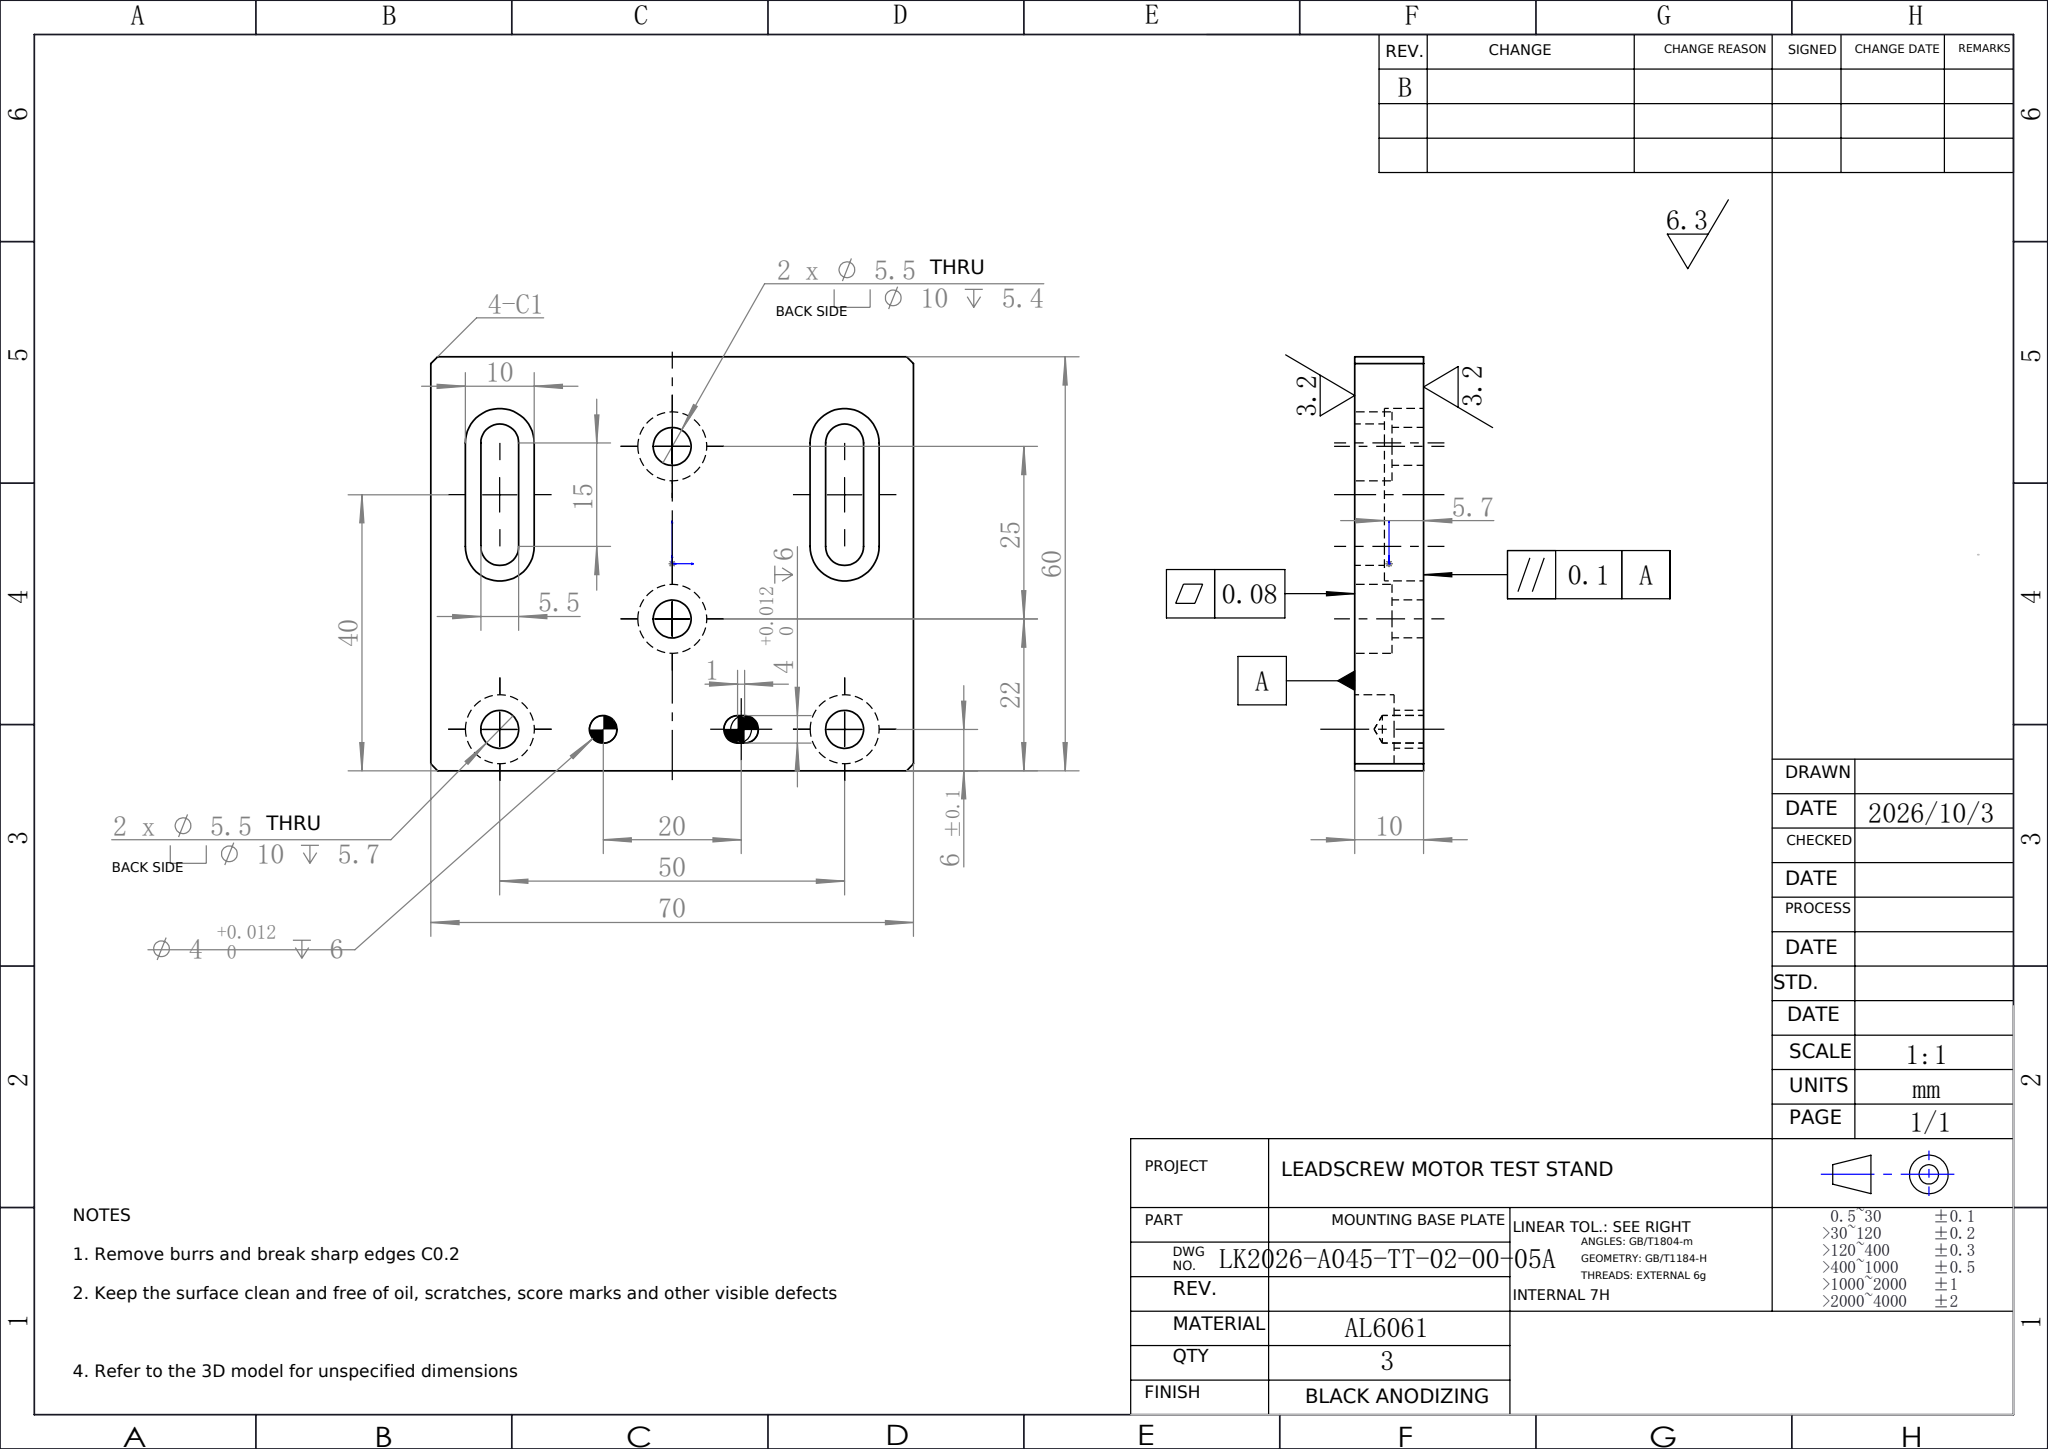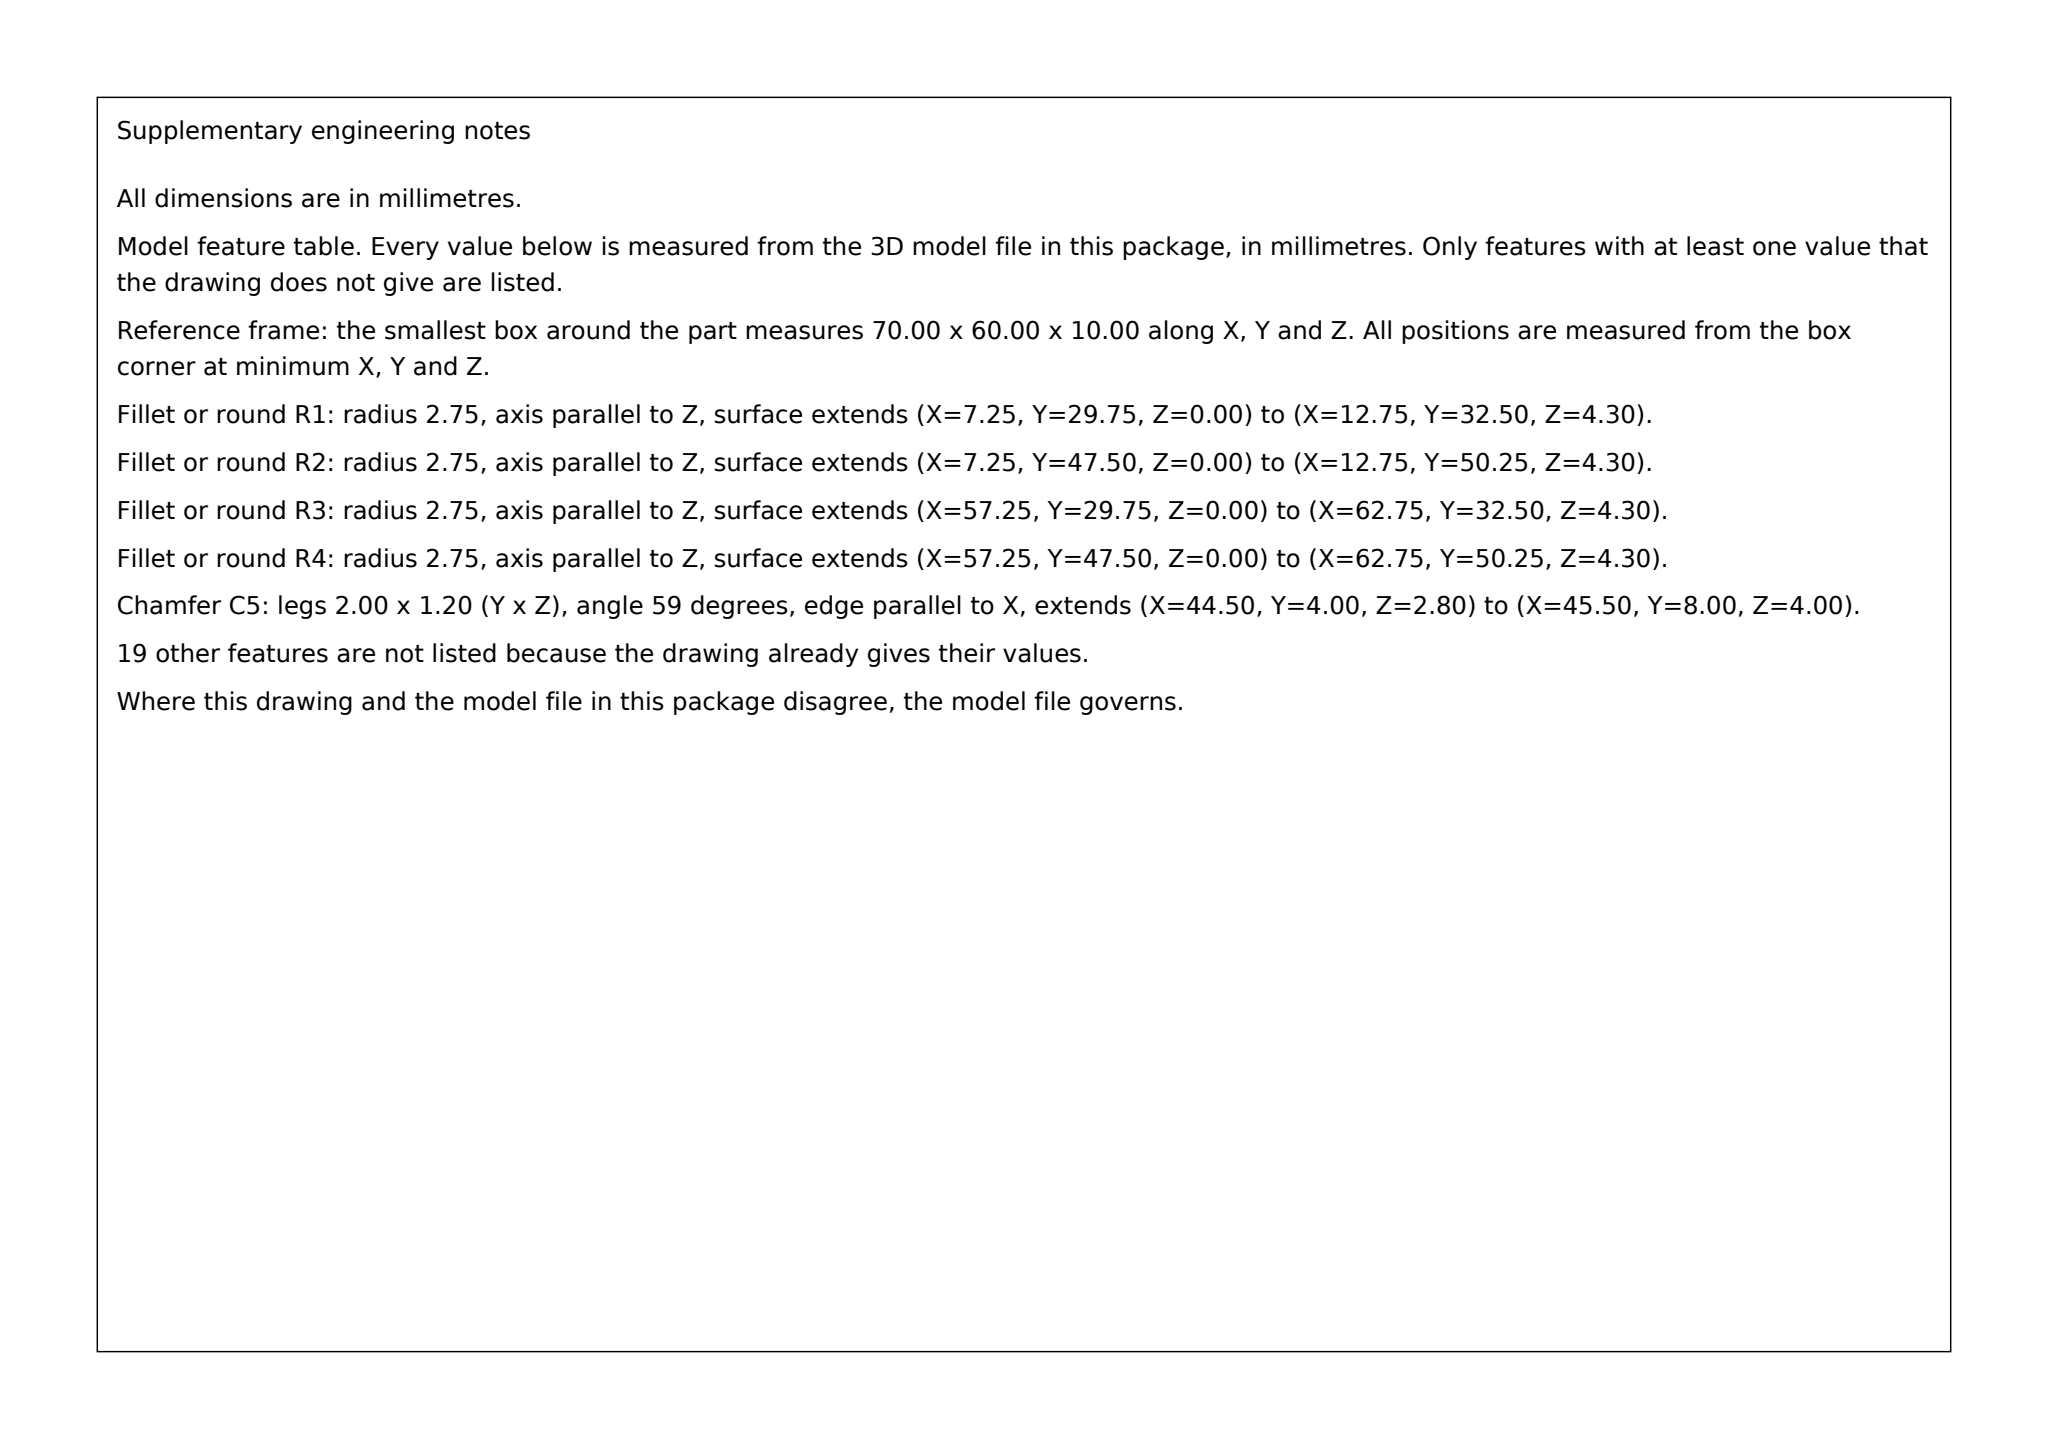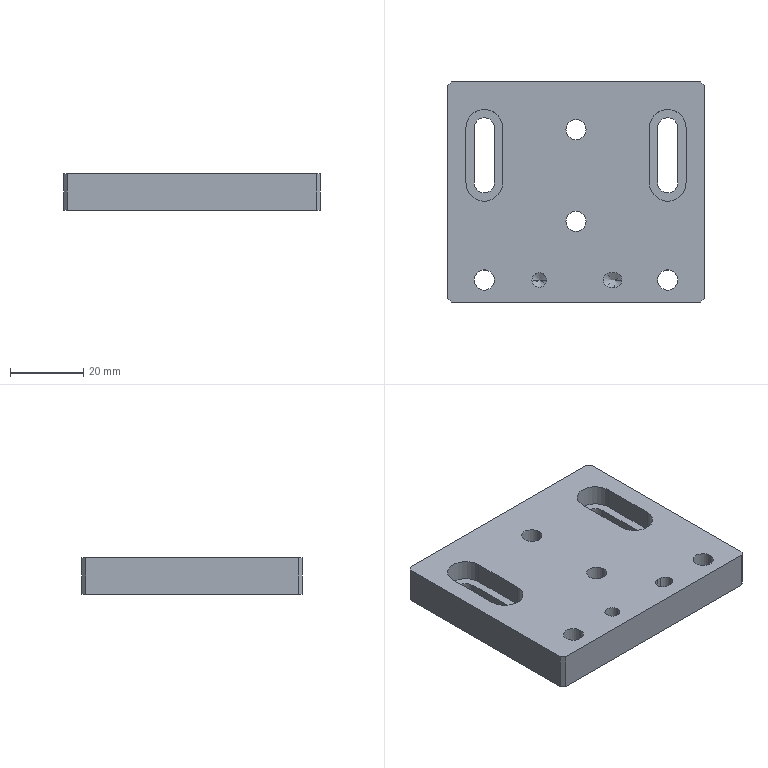Part | SolidWorks | mm | 1 solid | 62 faces | box 70 x 60 x 10 mm | volume 36107 mm3 | cylinder 29 | plane 28 | cone 5 | commonest cylinder face diameters 10 x12 5.5 x12 4 x5